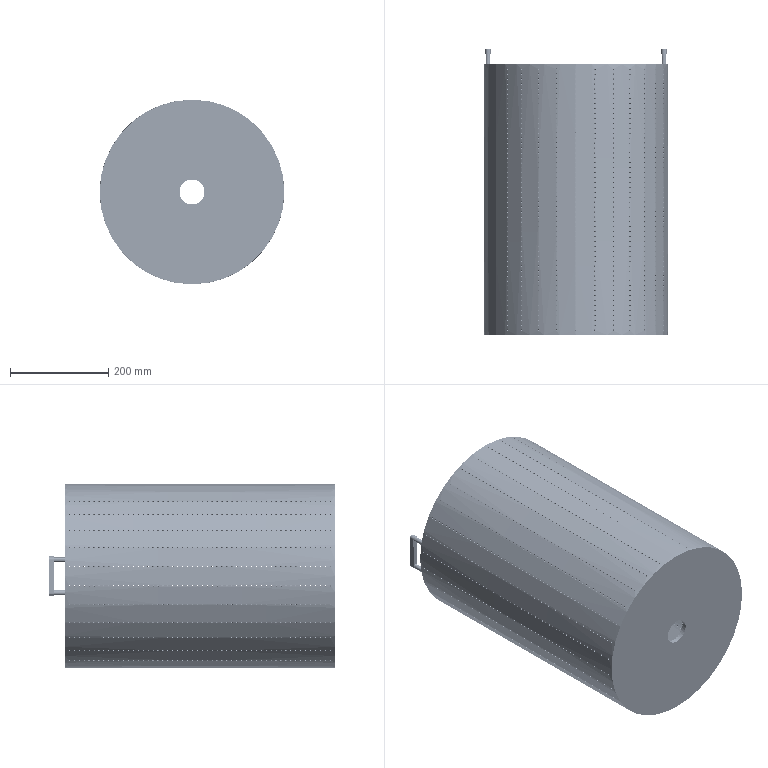Component | SolidWorks | FilterScreen-1 | 1 solid | 3300 faces | volume 7163322 mm3 | cylinder 3260 | plane 40 | commonest cylinder face diameters 3 x3240 9.256 x8 11.172 x6 51 x2 354.772 x2 374.772 x2